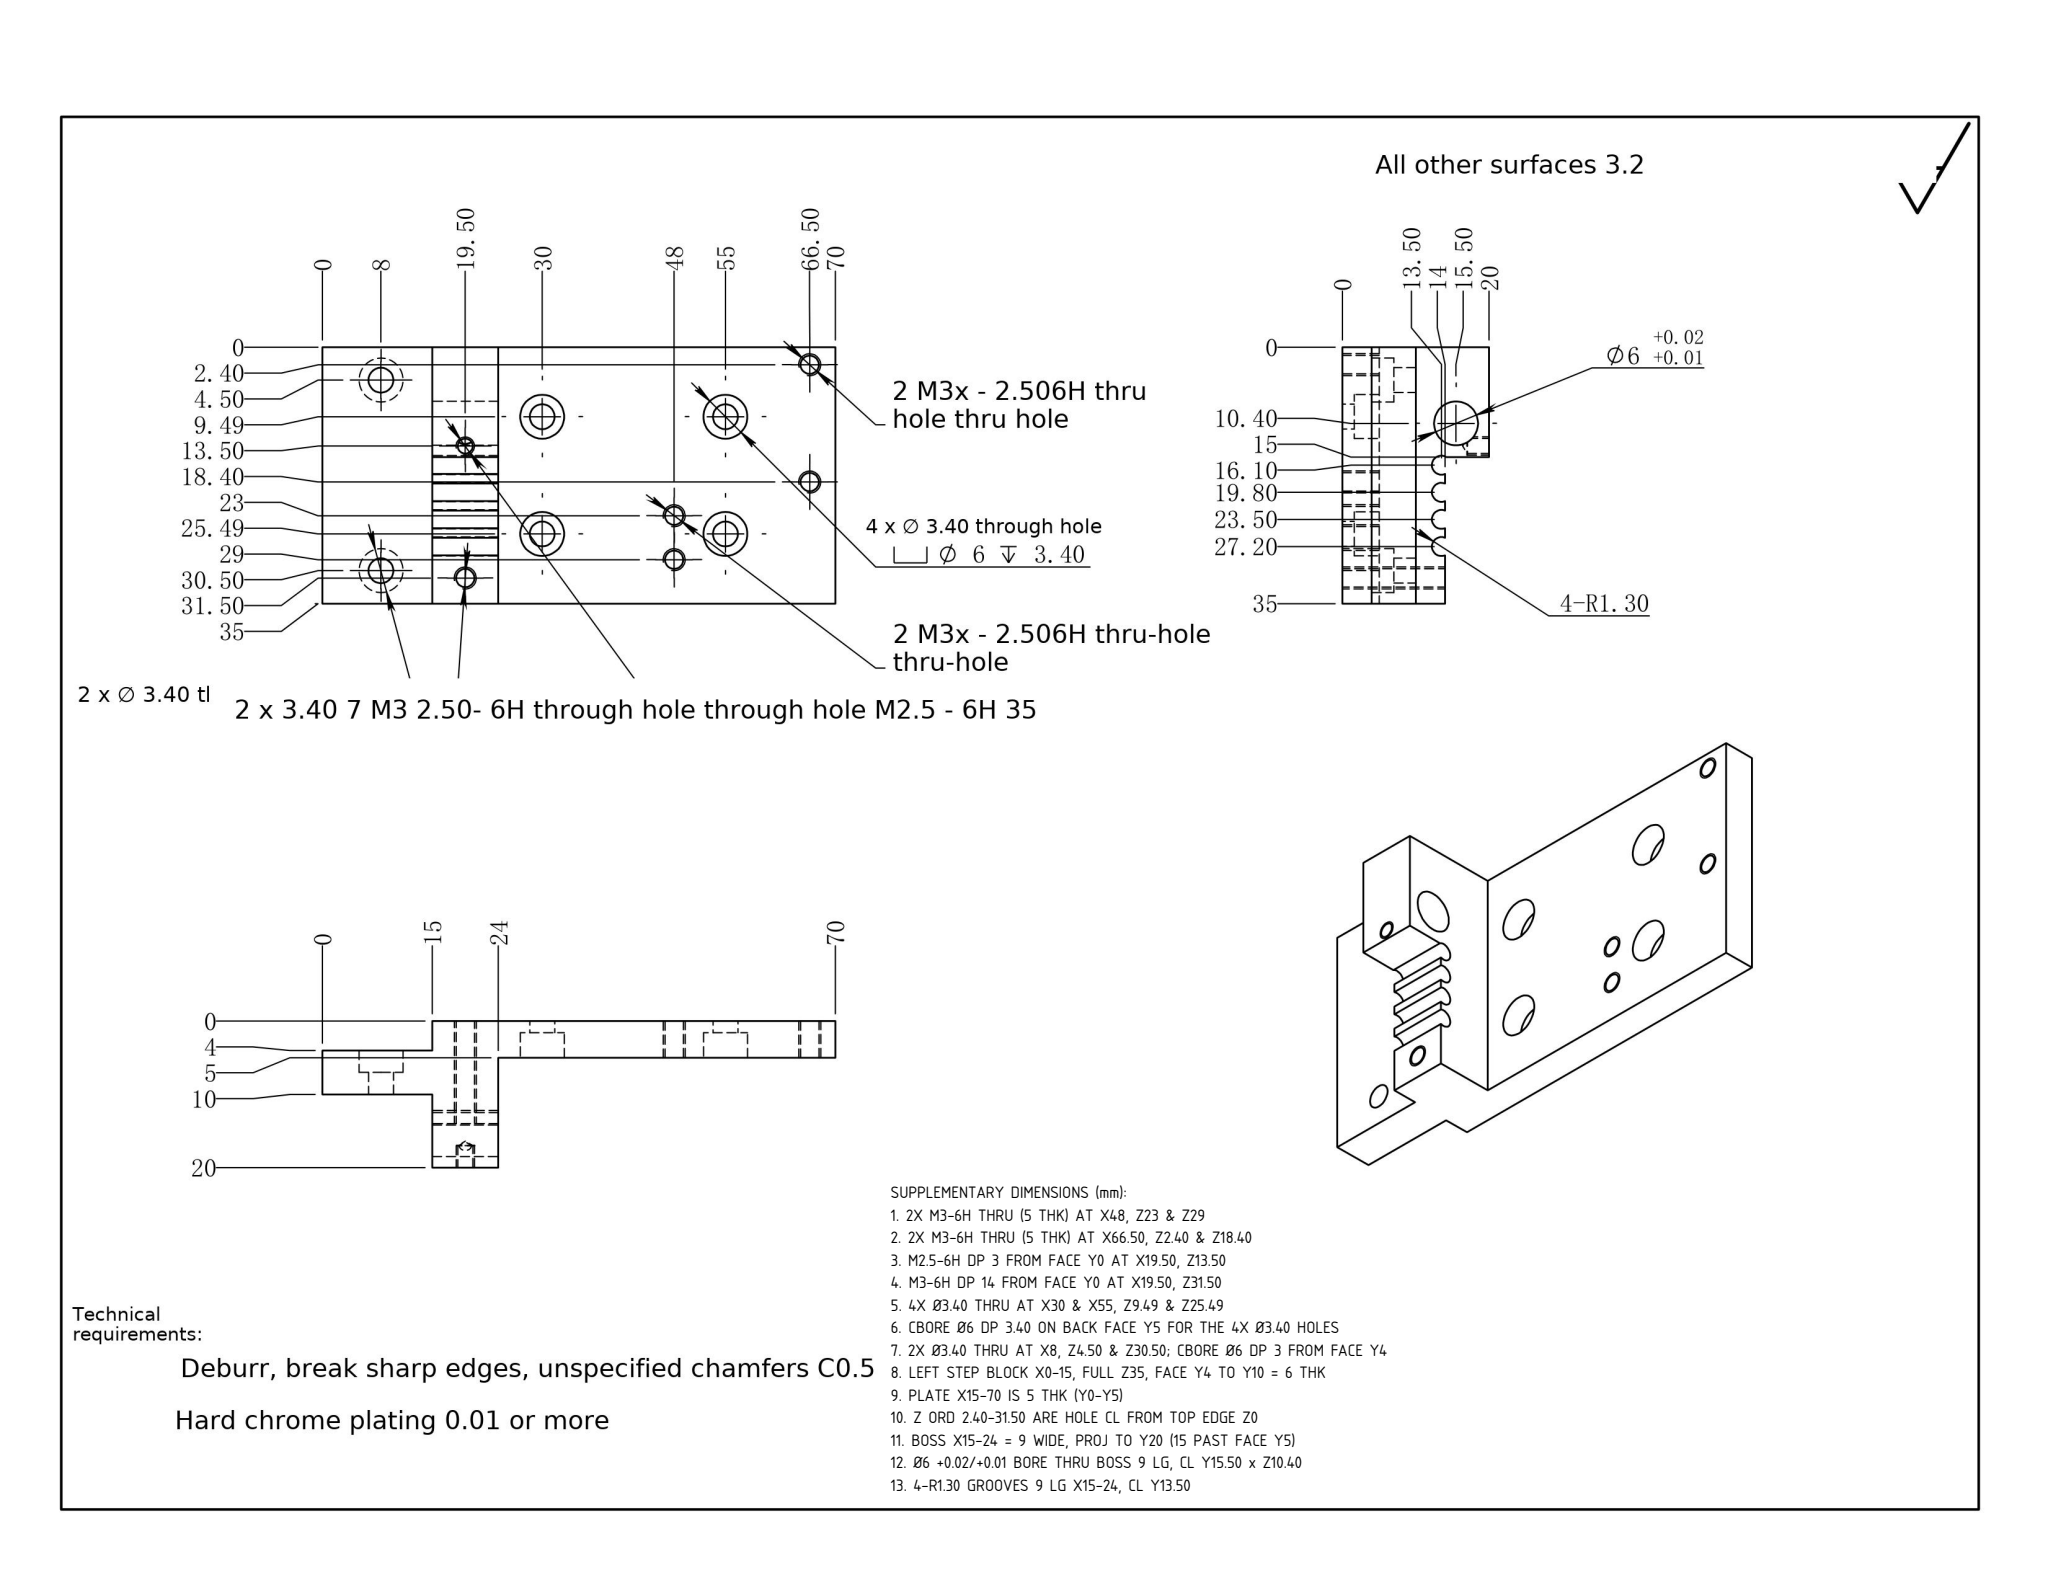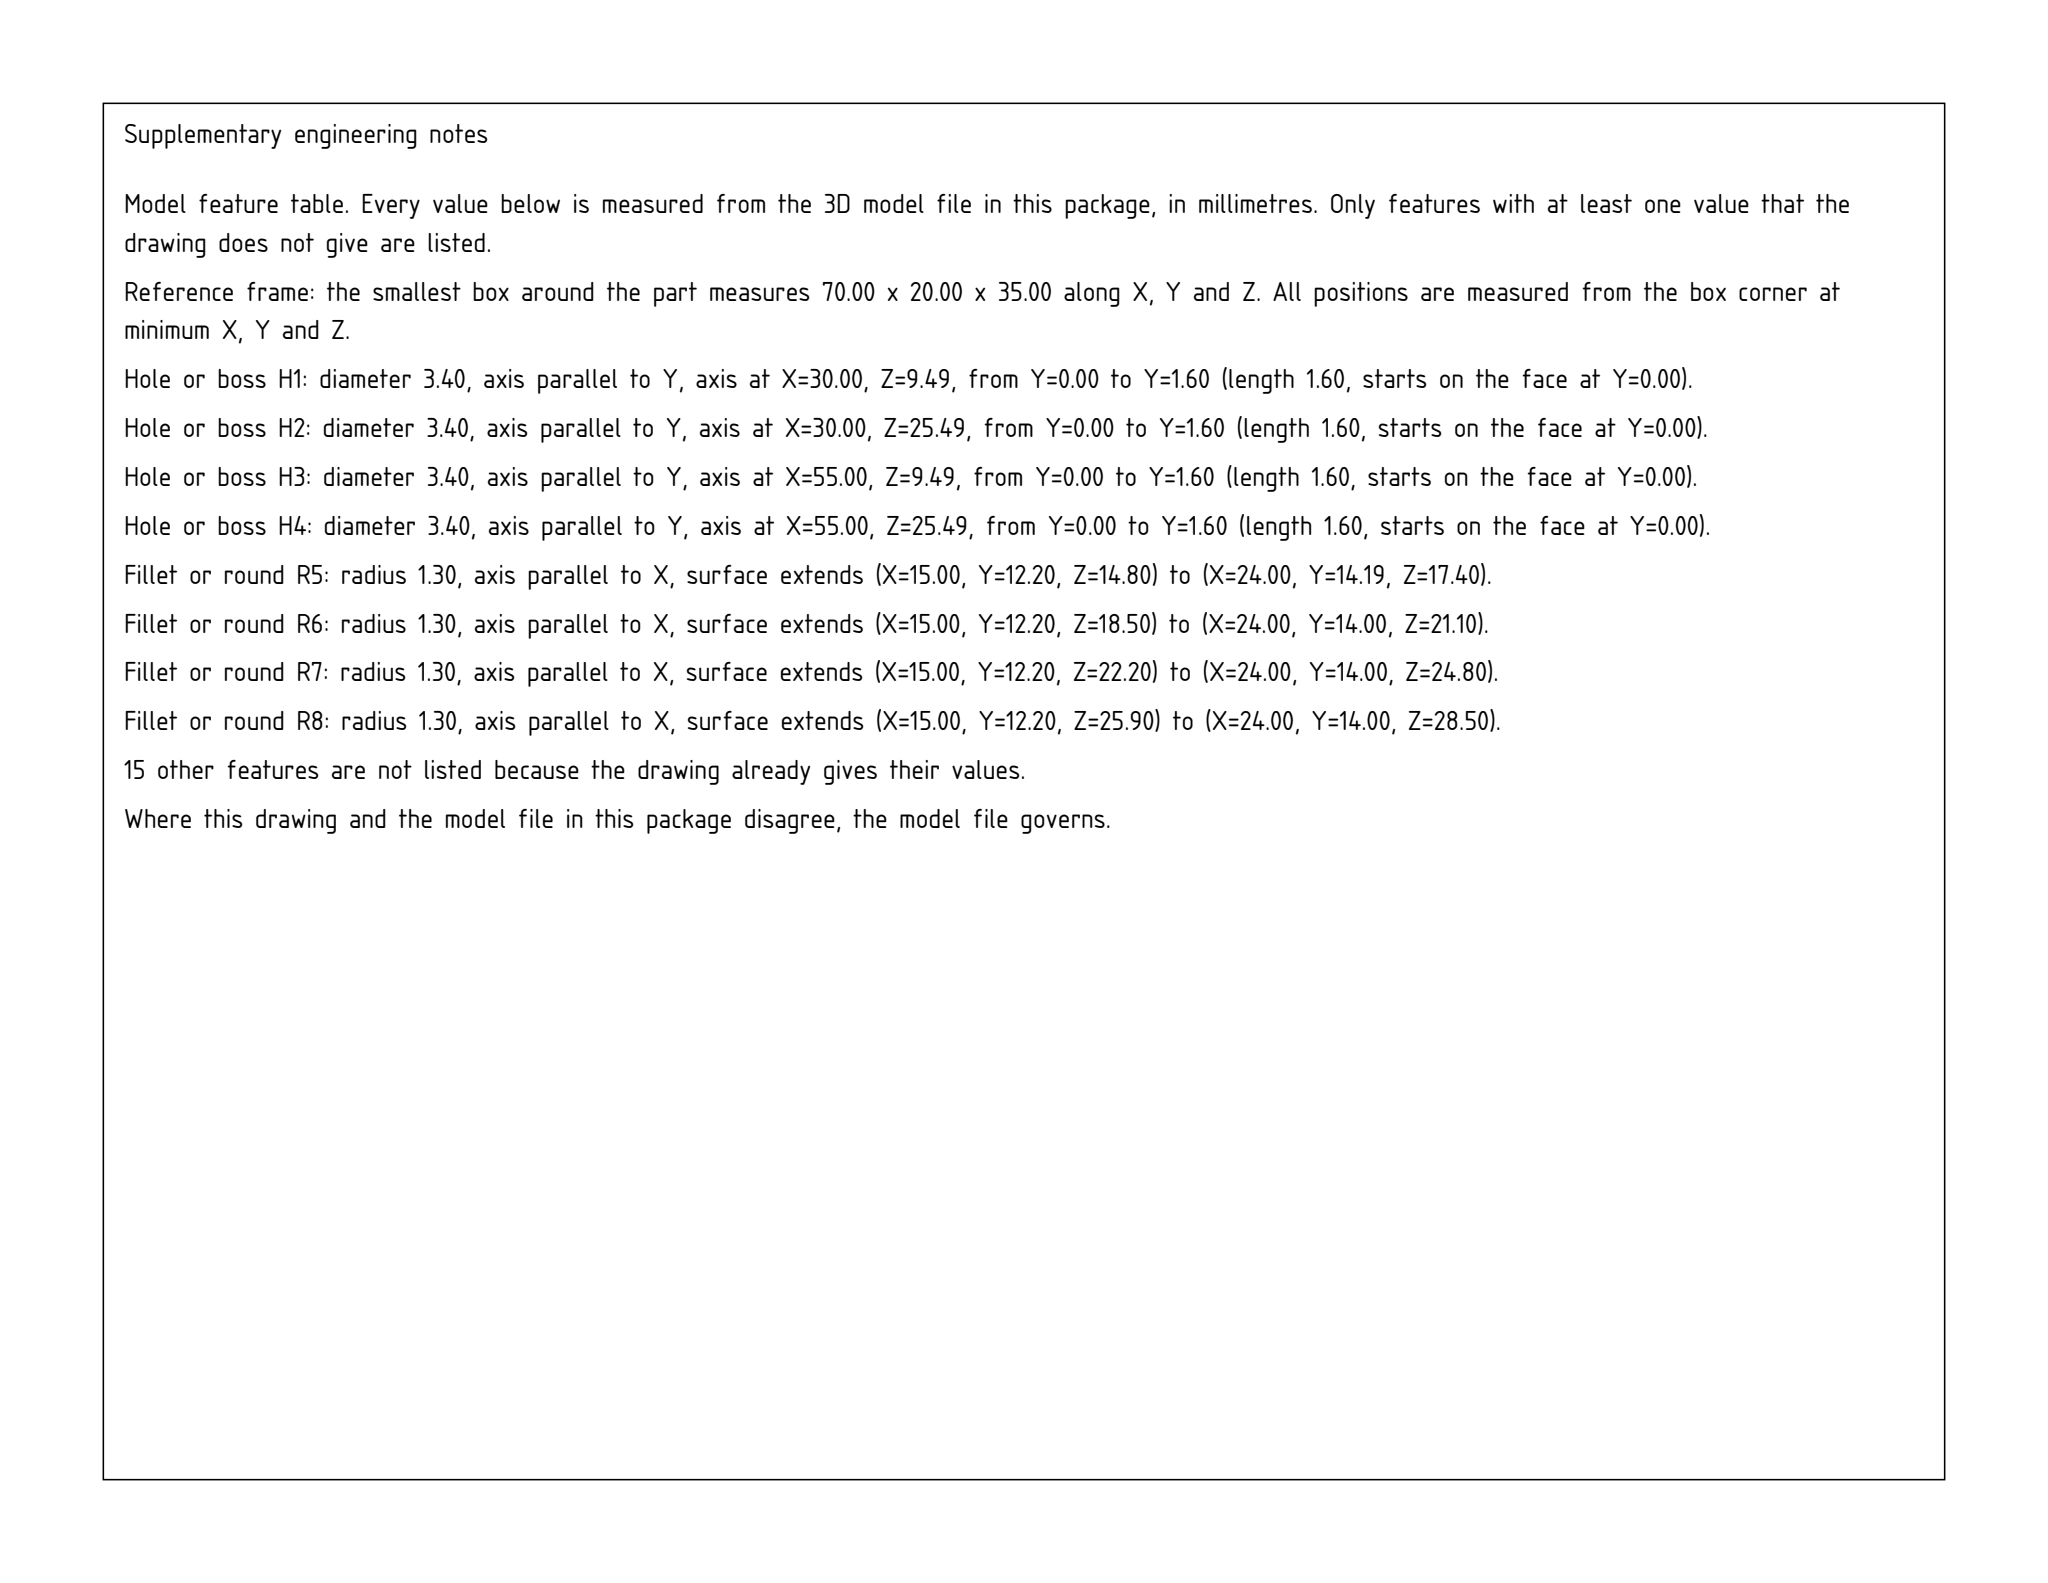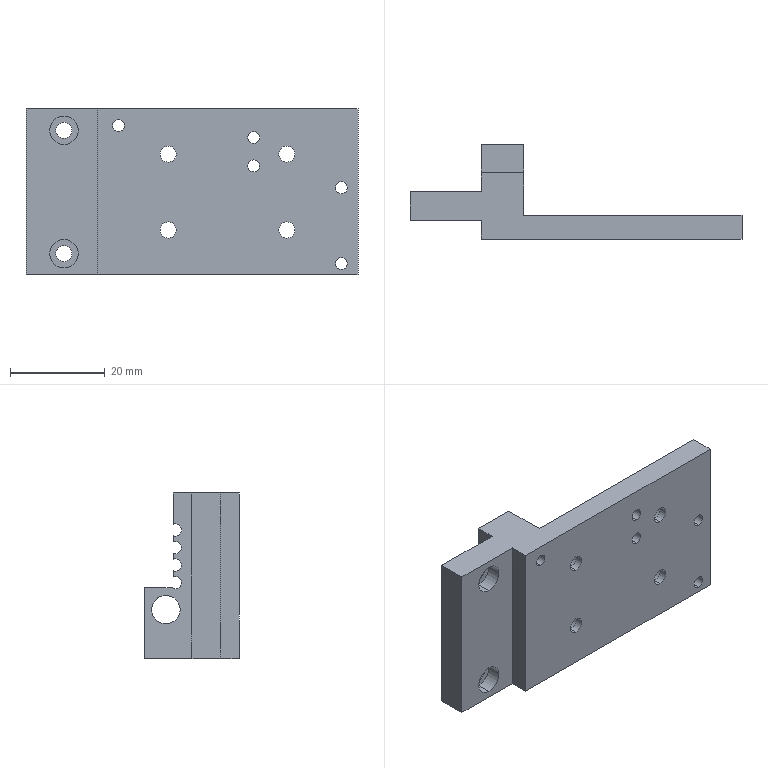Part | SolidWorks | mm | 1 solid | 67 faces | box 70 x 20 x 35 mm | volume 15180 mm3 | cylinder 42 | plane 23 | cone 2 | commonest cylinder face diameters 6 x14 3.4 x12 2.5 x10 2.6 x4 2.05 x2
build123d program:
from build123d import *

# Parameters (mm, degrees)
SKETCH2_W                                       = 70
SKETCH2_H                                       = 35
BOSS_EXTRUDE1_DEPTH                             = 20
SKETCH4_W                                       = 46
SKETCH4_H                                       = 15
CUT_EXTRUDE1_DEPTH                              = 54.385
SKETCH5_W                                       = 15
SKETCH5_H                                       = 10
CUT_EXTRUDE2_DEPTH                              = 54.385
SKETCH6_W                                       = 9
SKETCH6_H                                       = 20
CUT_EXTRUDE3_DEPTH                              = 6
M3_HEX_SOCKET_HEAD_CAP_SCREW_CBORE1_D           = 3.4
M3_HEX_SOCKET_HEAD_CAP_SCREW_CBORE1_CBORE_D     = 6
M3_HEX_SOCKET_HEAD_CAP_SCREW_CBORE1_CBORE_DEPTH = 3.4
M3_HEX_SOCKET_HEAD_CAP_SCREW_CBORE2_D           = 3.4
M3_HEX_SOCKET_HEAD_CAP_SCREW_CBORE2_CBORE_D     = 6
M3_HEX_SOCKET_HEAD_CAP_SCREW_CBORE2_CBORE_DEPTH = 7
SKETCH13_R                                      = 1.3
CUT_EXTRUDE4_DEPTH                              = 54.125
M3_TAPPED_HOLE1_D                               = 2.5
M3_TAPPED_HOLE2_D                               = 2.5
SKETCH18_R                                      = 3
CUT_EXTRUDE5_DEPTH                              = 54.125
M3_TAPPED_HOLE3_D                               = 2.5
M2_5_TAPPED_HOLE1_D                             = 2.05
M2_5_TAPPED_HOLE1_DEPTH                         = 3
M2_5_TAPPED_HOLE1_TIP                           = 0.6159
SKETCH25_W                                      = 15
SKETCH25_H                                      = 4
CUT_EXTRUDE6_DEPTH                              = 54.385


with BuildPart() as part:
    # Sketch2 → Boss-Extrude1 (new body)
    with BuildSketch(Plane(origin=(0, 0, 0), x_dir=(1, 0, 0), z_dir=(0, 1, 0))):
        Rectangle(SKETCH2_W, SKETCH2_H)
    extrude(amount=BOSS_EXTRUDE1_DEPTH)

    # Sketch4 → Cut-Extrude1 (cut, through all)
    with BuildSketch(Plane.XY.offset(17.5)):
        with Locations((12, 12.5)):
            Rectangle(SKETCH4_W, SKETCH4_H)
    extrude(amount=-CUT_EXTRUDE1_DEPTH, mode=Mode.SUBTRACT)

    # Sketch5 → Cut-Extrude2 (cut, through all)
    with BuildSketch(Plane.XY.offset(17.5)):
        with Locations((-27.5, 15)):
            Rectangle(SKETCH5_W, SKETCH5_H)
    extrude(amount=-CUT_EXTRUDE2_DEPTH, mode=Mode.SUBTRACT)

    # Sketch6 → Cut-Extrude3 (cut)
    with BuildSketch(Plane(origin=(0, 20, 0), x_dir=(1, 0, 0), z_dir=(0, 1, 0))):
        with Locations((-15.5, -7.5)):
            Rectangle(SKETCH6_W, SKETCH6_H)
    extrude(amount=-CUT_EXTRUDE3_DEPTH, mode=Mode.SUBTRACT)

    # M3 Hex Socket Head Cap Screw CBORE1 (through all)
    with Locations(Plane(origin=(0, 5, 0), x_dir=(1, 0, 0), z_dir=(0, 1, 0))):
        with Locations((-5, 8.015), (-5, -7.985), (20, -7.985), (20, 8.015)):
            CounterBoreHole(M3_HEX_SOCKET_HEAD_CAP_SCREW_CBORE1_D / 2, M3_HEX_SOCKET_HEAD_CAP_SCREW_CBORE1_CBORE_D / 2, M3_HEX_SOCKET_HEAD_CAP_SCREW_CBORE1_CBORE_DEPTH)

    # M3 Hex Socket Head Cap Screw CBORE2 (through all)
    with Locations(Plane(origin=(0, 0, 0), x_dir=(-1, 0, 0), z_dir=(0, -1, 0))):
        with Locations((27, 13), (27, -13)):
            CounterBoreHole(M3_HEX_SOCKET_HEAD_CAP_SCREW_CBORE2_D / 2, M3_HEX_SOCKET_HEAD_CAP_SCREW_CBORE2_CBORE_D / 2, M3_HEX_SOCKET_HEAD_CAP_SCREW_CBORE2_CBORE_DEPTH)

    # Sketch13 → Cut-Extrude4 (cut, through all)
    with BuildSketch(Plane(origin=(-11, 0, 0), x_dir=(0, 0, -1), z_dir=(1, 0, 0))):
        with Locations((-9.7, 13.5)):
            Circle(SKETCH13_R)
        with Locations((-6, 13.5)):
            Circle(SKETCH13_R)
        with Locations((-2.3, 13.5)):
            Circle(SKETCH13_R)
        with Locations((1.4, 13.5)):
            Circle(SKETCH13_R)
    extrude(amount=-CUT_EXTRUDE4_DEPTH, mode=Mode.SUBTRACT)

    # M3 Tapped Hole1 (through all)
    with Locations(Plane(origin=(0, 5, 0), x_dir=(1, 0, 0), z_dir=(0, 1, 0))):
        with Locations((13, -5.5), (13, -11.5)):
            Hole(M3_TAPPED_HOLE1_D / 2)

    # M3 Tapped Hole2 (through all)
    with Locations(Plane(origin=(0, 14, 0), x_dir=(1, 0, 0), z_dir=(0, 1, 0))):
        with Locations((-15.5, -14)):
            Hole(M3_TAPPED_HOLE2_D / 2)

    # Sketch18 → Cut-Extrude5 (cut, through all)
    with BuildSketch(Plane(origin=(-11, 0, 0), x_dir=(0, 0, -1), z_dir=(1, 0, 0))):
        with Locations(Location((7.1, 15.5, 0), (0, 0, 90))):
            Circle(SKETCH18_R)
    extrude(amount=-CUT_EXTRUDE5_DEPTH, mode=Mode.SUBTRACT)

    # M3 Tapped Hole3 (through all)
    with Locations(Plane(origin=(0, 5, 0), x_dir=(1, 0, 0), z_dir=(0, 1, 0))):
        with Locations((31.5, 15.1), (31.5, -0.9)):
            Hole(M3_TAPPED_HOLE3_D / 2)

    # M2.5 Tapped Hole1
    with Locations(Plane(origin=(0, 20, 0), x_dir=(1, 0, 0), z_dir=(0, 1, 0))):
        with Locations((-15.5, 4)):
            Hole(M2_5_TAPPED_HOLE1_D / 2, depth=M2_5_TAPPED_HOLE1_DEPTH)
            with Locations((0, 0, -(M2_5_TAPPED_HOLE1_DEPTH + M2_5_TAPPED_HOLE1_TIP / 2))):  # 118° drill point
                Cone(0, M2_5_TAPPED_HOLE1_D / 2, M2_5_TAPPED_HOLE1_TIP, mode=Mode.SUBTRACT)

    # Sketch25 → Cut-Extrude6 (cut, through all)
    with BuildSketch(Plane.XY.offset(17.5)):
        with Locations((-27.5, 2)):
            Rectangle(SKETCH25_W, SKETCH25_H)
    extrude(amount=-CUT_EXTRUDE6_DEPTH, mode=Mode.SUBTRACT)


solid = part.part